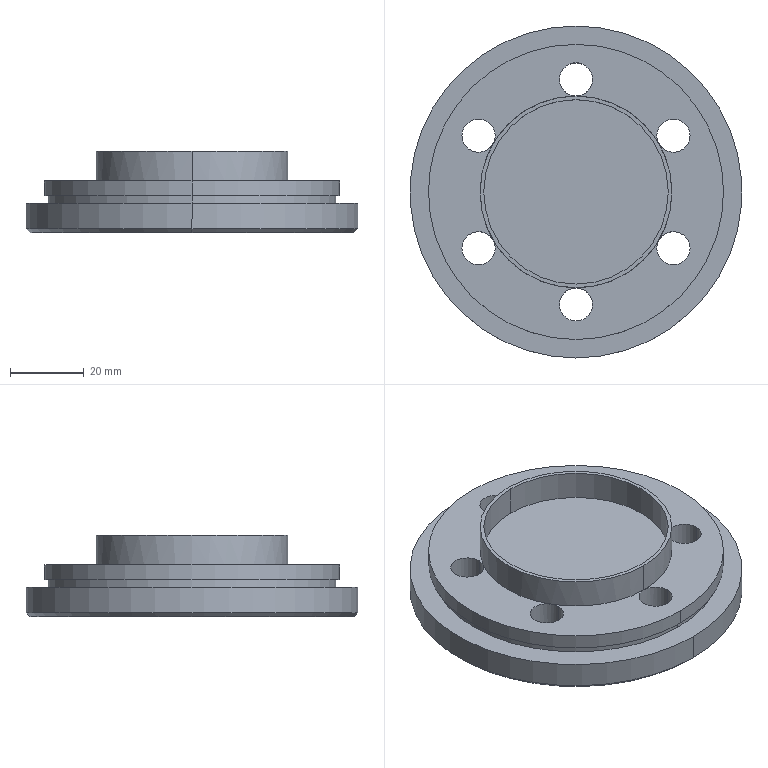Component | SolidWorks | SecondaryEndCover-2 | 1 solid | 33 faces | box 90 x 90 x 22 mm | volume 75360 mm3 | cylinder 22 | plane 7 | cone 2 | torus 2 | commonest cylinder face diameters 9 x12 50 x2 52 x2 78 x2 90 x2 80 x2
build123d program:
from build123d import *

# Parameters (mm, degrees)
SKETCH2_R                  = 26
BOSS_EXTRUDE1_DEPTH        = 8
F_8_5_8_5_DIAMETER_HOLE1_D = 9
CIRPATTERN2_COUNT          = 6
CHAMFER1_SIZE              = 1
SKETCH8_R                  = 25
CUT_EXTRUDE1_DEPTH         = 8


with BuildPart() as part:
    # Sketch1 → Revolve1 (revolve)
    with BuildSketch(Plane(origin=(0, 0, 0), x_dir=(-1, 0, 0), z_dir=(0, 0, -1)), mode=Mode.PRIVATE) as revolve1_sk:
        Polygon((-6, 40), (-6, 0), (8, 0), (8, 45), (0, 45), (0, 39), (-2, 39), (-2, 40), align=None)
    revolve(revolve1_sk.sketch.rotate(Axis((6, 0, 0), (-1, 0, 0)), 180), axis=Axis((6, 0, 0), (-1, 0, 0)))

    # Sketch2 → Boss-Extrude1 (add)
    with BuildSketch(Plane(origin=(6, 0, 0), x_dir=(0, 0, -1), z_dir=(1, 0, 0))):
        with Locations(Location((0, 0, 0), (0, 0, 90))):
            Circle(SKETCH2_R)
    extrude(amount=BOSS_EXTRUDE1_DEPTH)

    # Sketch5 → Cut-Revolve2 (revolve, cut)
    with BuildSketch(Plane(origin=(0, 0, 0), x_dir=(-1, 0, 0), z_dir=(0, 0, -1)), mode=Mode.PRIVATE) as cut_revolve2_sk:
        with BuildLine():
            Line((7, 17), (7, 0))
            Line((7, 0), (8, 0))
            Line((8, 0), (8, 18))
            ThreePointArc((8, 18), (7.293, 17.707), (7, 17))
        make_face()
    revolve(cut_revolve2_sk.sketch.rotate(Axis((-4.998, 0, 0), (-1, 0, 0)), 180), axis=Axis((-4.998, 0, 0), (-1, 0, 0)), mode=Mode.SUBTRACT)

    # 8.5 _8.5_ Diameter Hole1 (through all)
    with Locations(Plane.ZY.offset(8)):
        with Locations((0, 30.5)):
            f_8_5_8_5_diameter_hole1 = Hole(F_8_5_8_5_DIAMETER_HOLE1_D / 2)

    # CirPattern2: 8.5 _8.5_ Diameter Hole1 ×6 about axis
    cirpattern2_axis = Axis((0, 0, 0), (1, 0, 0))
    for i in range(1, CIRPATTERN2_COUNT):
        add(f_8_5_8_5_diameter_hole1.rotate(cirpattern2_axis, i * 360 / CIRPATTERN2_COUNT), mode=Mode.SUBTRACT)

    # Chamfer1
    chamfer1_edges = [part.edges().sort_by_distance(p)[0] for p in [
        (-8, 45, 0),
    ]]
    chamfer(chamfer1_edges, length=CHAMFER1_SIZE)

    # Sketch8 → Cut-Extrude1 (cut)
    with BuildSketch(Plane(origin=(14, 0, 0), x_dir=(0, 0, -1), z_dir=(1, 0, 0))):
        with Locations(Location((0, 0, 0), (0, 0, 90))):
            Circle(SKETCH8_R)
    extrude(amount=-CUT_EXTRUDE1_DEPTH, mode=Mode.SUBTRACT)


solid = part.part

# Placed as in the assembly
solid = solid.moved(Location((-225, 0, -153), (0, -90, 0)))
STEP:
#1=COLOUR_RGB('',0.7922,0.8196,0.9333);
#2=FILL_AREA_STYLE_COLOUR('',#1);
#3=FILL_AREA_STYLE('',(#2));
#4=SURFACE_STYLE_FILL_AREA(#3);
#5=SURFACE_SIDE_STYLE('',(#4));
#6=SURFACE_STYLE_USAGE(.BOTH.,#5);
#7=PRESENTATION_STYLE_ASSIGNMENT((#6));
#8=CARTESIAN_POINT('',(-8.858,-0.9843,-5.787));
#9=VERTEX_POINT('',#8);
#10=CARTESIAN_POINT('',(-8.858,0.9843,-5.787));
#11=VERTEX_POINT('',#10);
#12=CARTESIAN_POINT('',(-8.858,-0.,-5.787));
#13=DIRECTION('',(0.,-0.,1.));
#14=DIRECTION('',(0.,1.,0.));
#15=AXIS2_PLACEMENT_3D('',#12,#13,#14);
#16=CIRCLE('',#15,0.9843);
#17=EDGE_CURVE('',#9,#11,#16,.T.);
#18=ORIENTED_EDGE('',*,*,#17,.F.);
#19=CARTESIAN_POINT('',(-8.858,-0.9843,-5.472));
#20=VERTEX_POINT('',#19);
#21=CARTESIAN_POINT('',(-8.858,-0.9843,-5.787));
#22=DIRECTION('',(0.,-0.,1.));
#23=VECTOR('',#22,39.37);
#24=LINE('',#21,#23);
#25=EDGE_CURVE('',#9,#20,#24,.T.);
#26=ORIENTED_EDGE('',*,*,#25,.T.);
#27=CARTESIAN_POINT('',(-8.858,0.9843,-5.472));
#28=VERTEX_POINT('',#27);
#29=CARTESIAN_POINT('',(-8.858,-0.,-5.472));
#30=DIRECTION('',(0.,-0.,1.));
#31=DIRECTION('',(0.,1.,0.));
#32=AXIS2_PLACEMENT_3D('',#29,#30,#31);
#33=CIRCLE('',#32,0.9843);
#34=EDGE_CURVE('',#20,#28,#33,.T.);
#35=ORIENTED_EDGE('',*,*,#34,.T.);
#36=CARTESIAN_POINT('',(-8.858,0.9843,-5.787));
#37=DIRECTION('',(0.,-0.,1.));
#38=VECTOR('',#37,39.37);
#39=LINE('',#36,#38);
#40=EDGE_CURVE('',#11,#28,#39,.T.);
#41=ORIENTED_EDGE('',*,*,#40,.F.);
#42=EDGE_LOOP('',(#18,#26,#35,#41));
#43=FACE_OUTER_BOUND('',#42,.T.);
#44=CARTESIAN_POINT('',(-8.858,-0.,-5.787));
#45=DIRECTION('',(0.,-0.,1.));
#46=DIRECTION('',(0.,1.,0.));
#47=AXIS2_PLACEMENT_3D('',#44,#45,#46);
#48=CYLINDRICAL_SURFACE('',#47,0.9843);
#49=ADVANCED_FACE('',(#43),#48,.F.);
#50=CARTESIAN_POINT('',(-8.858,-1.732,-6.339));
#51=VERTEX_POINT('',#50);
#52=CARTESIAN_POINT('',(-8.858,1.732,-6.339));
#53=VERTEX_POINT('',#52);
#54=CARTESIAN_POINT('',(-8.858,-0.,-6.339));
#55=DIRECTION('',(-0.,0.,-1.));
#56=DIRECTION('',(0.,-1.,0.));
#57=AXIS2_PLACEMENT_3D('',#54,#55,#56);
#58=CIRCLE('',#57,1.732);
#59=EDGE_CURVE('',#51,#53,#58,.T.);
#60=ORIENTED_EDGE('',*,*,#59,.F.);
#61=CARTESIAN_POINT('',(-8.858,-1.772,-6.299));
#62=VERTEX_POINT('',#61);
#63=CARTESIAN_POINT('',(-8.858,-1.732,-6.339));
#64=DIRECTION('',(0.,-0.7071,0.7071));
#65=VECTOR('',#64,39.37);
#66=LINE('',#63,#65);
#67=EDGE_CURVE('',#51,#62,#66,.T.);
#68=ORIENTED_EDGE('',*,*,#67,.T.);
#69=CARTESIAN_POINT('',(-8.858,1.772,-6.299));
#70=VERTEX_POINT('',#69);
#71=CARTESIAN_POINT('',(-8.858,-0.,-6.299));
#72=DIRECTION('',(0.,-0.,1.));
#73=DIRECTION('',(0.,-1.,0.));
#74=AXIS2_PLACEMENT_3D('',#71,#72,#73);
#75=CIRCLE('',#74,1.772);
#76=EDGE_CURVE('',#70,#62,#75,.T.);
#77=ORIENTED_EDGE('',*,*,#76,.F.);
#78=CARTESIAN_POINT('',(-8.858,1.732,-6.339));
#79=DIRECTION('',(0.,0.7071,0.7071));
#80=VECTOR('',#79,39.37);
#81=LINE('',#78,#80);
#82=EDGE_CURVE('',#53,#70,#81,.T.);
#83=ORIENTED_EDGE('',*,*,#82,.F.);
#84=EDGE_LOOP('',(#60,#68,#77,#83));
#85=FACE_OUTER_BOUND('',#84,.T.);
#86=CARTESIAN_POINT('',(-8.858,-0.,-6.339));
#87=DIRECTION('',(0.,-0.,1.));
#88=DIRECTION('',(0.,1.,0.));
#89=AXIS2_PLACEMENT_3D('',#86,#87,#88);
#90=CONICAL_SURFACE('',#89,1.732,0.7854);
#91=ADVANCED_FACE('',(#85),#90,.T.);
#92=CARTESIAN_POINT('',(-9.745,0.5118,-5.787));
#93=VERTEX_POINT('',#92);
#94=CARTESIAN_POINT('',(-9.721,0.6004,-5.787));
#95=VERTEX_POINT('',#94);
#96=CARTESIAN_POINT('',(-9.898,0.6004,-5.787));
#97=DIRECTION('',(0.,-0.,1.));
#98=DIRECTION('',(0.,1.,0.));
#99=AXIS2_PLACEMENT_3D('',#96,#97,#98);
#100=CIRCLE('',#99,0.1772);
#101=EDGE_CURVE('',#93,#95,#100,.T.);
#102=ORIENTED_EDGE('',*,*,#101,.T.);
#103=CARTESIAN_POINT('',(-9.721,0.6004,-6.339));
#104=VERTEX_POINT('',#103);
#105=CARTESIAN_POINT('',(-9.721,0.6004,-6.339));
#106=DIRECTION('',(-0.,0.,-1.));
#107=VECTOR('',#106,39.37);
#108=LINE('',#105,#107);
#109=EDGE_CURVE('',#95,#104,#108,.T.);
#110=ORIENTED_EDGE('',*,*,#109,.T.);
#111=CARTESIAN_POINT('',(-10.075,0.6004,-6.339));
#112=VERTEX_POINT('',#111);
#113=CARTESIAN_POINT('',(-9.898,0.6004,-6.339));
#114=DIRECTION('',(-0.,0.,-1.));
#115=DIRECTION('',(-1.,0.,0.));
#116=AXIS2_PLACEMENT_3D('',#113,#114,#115);
#117=CIRCLE('',#116,0.1772);
#118=EDGE_CURVE('',#104,#112,#117,.T.);
#119=ORIENTED_EDGE('',*,*,#118,.T.);
#120=CARTESIAN_POINT('',(-10.075,0.6004,-5.787));
#121=VERTEX_POINT('',#120);
#122=CARTESIAN_POINT('',(-10.075,0.6004,-6.339));
#123=DIRECTION('',(-0.,0.,-1.));
#124=VECTOR('',#123,39.37);
#125=LINE('',#122,#124);
#126=EDGE_CURVE('',#121,#112,#125,.T.);
#127=ORIENTED_EDGE('',*,*,#126,.F.);
#128=CARTESIAN_POINT('',(-9.898,0.6004,-5.787));
#129=DIRECTION('',(0.,-0.,1.));
#130=DIRECTION('',(0.,1.,0.));
#131=AXIS2_PLACEMENT_3D('',#128,#129,#130);
#132=CIRCLE('',#131,0.1772);
#133=EDGE_CURVE('',#121,#93,#132,.T.);
#134=ORIENTED_EDGE('',*,*,#133,.T.);
#135=EDGE_LOOP('',(#102,#110,#119,#127,#134));
#136=FACE_OUTER_BOUND('',#135,.T.);
#137=CARTESIAN_POINT('',(-9.898,0.6004,-6.339));
#138=DIRECTION('',(-0.,0.,-1.));
#139=DIRECTION('',(-1.,0.,0.));
#140=AXIS2_PLACEMENT_3D('',#137,#138,#139);
#141=CYLINDRICAL_SURFACE('',#140,0.1772);
#142=ADVANCED_FACE('',(#136),#141,.F.);
#143=CARTESIAN_POINT('',(-10.075,-0.6004,-5.787));
#144=VERTEX_POINT('',#143);
#145=CARTESIAN_POINT('',(-9.721,-0.6004,-5.787));
#146=VERTEX_POINT('',#145);
#147=CARTESIAN_POINT('',(-9.898,-0.6004,-5.787));
#148=DIRECTION('',(0.,-0.,1.));
#149=DIRECTION('',(0.,1.,0.));
#150=AXIS2_PLACEMENT_3D('',#147,#148,#149);
#151=CIRCLE('',#150,0.1772);
#152=EDGE_CURVE('',#144,#146,#151,.T.);
#153=ORIENTED_EDGE('',*,*,#152,.T.);
#154=CARTESIAN_POINT('',(-9.721,-0.6004,-6.339));
#155=VERTEX_POINT('',#154);
#156=CARTESIAN_POINT('',(-9.721,-0.6004,-6.339));
#157=DIRECTION('',(-0.,0.,-1.));
#158=VECTOR('',#157,39.37);
#159=LINE('',#156,#158);
#160=EDGE_CURVE('',#146,#155,#159,.T.);
#161=ORIENTED_EDGE('',*,*,#160,.T.);
#162=CARTESIAN_POINT('',(-10.075,-0.6004,-6.339));
#163=VERTEX_POINT('',#162);
#164=CARTESIAN_POINT('',(-9.898,-0.6004,-6.339));
#165=DIRECTION('',(-0.,0.,-1.));
#166=DIRECTION('',(-1.,0.,0.));
#167=AXIS2_PLACEMENT_3D('',#164,#165,#166);
#168=CIRCLE('',#167,0.1772);
#169=EDGE_CURVE('',#155,#163,#168,.T.);
#170=ORIENTED_EDGE('',*,*,#169,.T.);
#171=CARTESIAN_POINT('',(-10.075,-0.6004,-6.339));
#172=DIRECTION('',(-0.,0.,-1.));
#173=VECTOR('',#172,39.37);
#174=LINE('',#171,#173);
#175=EDGE_CURVE('',#144,#163,#174,.T.);
#176=ORIENTED_EDGE('',*,*,#175,.F.);
#177=EDGE_LOOP('',(#153,#161,#170,#176));
#178=FACE_OUTER_BOUND('',#177,.T.);
#179=CARTESIAN_POINT('',(-9.898,-0.6004,-6.339));
#180=DIRECTION('',(-0.,0.,-1.));
#181=DIRECTION('',(-1.,0.,0.));
#182=AXIS2_PLACEMENT_3D('',#179,#180,#181);
#183=CYLINDRICAL_SURFACE('',#182,0.1772);
#184=ADVANCED_FACE('',(#178),#183,.F.);
#185=CARTESIAN_POINT('',(-9.035,-1.201,-5.787));
#186=VERTEX_POINT('',#185);
#187=CARTESIAN_POINT('',(-8.681,-1.201,-5.787));
#188=VERTEX_POINT('',#187);
#189=CARTESIAN_POINT('',(-8.858,-1.201,-5.787));
#190=DIRECTION('',(0.,-0.,1.));
#191=DIRECTION('',(0.,1.,0.));
#192=AXIS2_PLACEMENT_3D('',#189,#190,#191);
#193=CIRCLE('',#192,0.1772);
#194=EDGE_CURVE('',#186,#188,#193,.T.);
#195=ORIENTED_EDGE('',*,*,#194,.T.);
#196=CARTESIAN_POINT('',(-8.681,-1.201,-6.339));
#197=VERTEX_POINT('',#196);
#198=CARTESIAN_POINT('',(-8.681,-1.201,-6.339));
#199=DIRECTION('',(-0.,0.,-1.));
#200=VECTOR('',#199,39.37);
#201=LINE('',#198,#200);
#202=EDGE_CURVE('',#188,#197,#201,.T.);
#203=ORIENTED_EDGE('',*,*,#202,.T.);
#204=CARTESIAN_POINT('',(-9.035,-1.201,-6.339));
#205=VERTEX_POINT('',#204);
#206=CARTESIAN_POINT('',(-8.858,-1.201,-6.339));
#207=DIRECTION('',(-0.,0.,-1.));
#208=DIRECTION('',(-1.,0.,0.));
#209=AXIS2_PLACEMENT_3D('',#206,#207,#208);
#210=CIRCLE('',#209,0.1772);
#211=EDGE_CURVE('',#197,#205,#210,.T.);
#212=ORIENTED_EDGE('',*,*,#211,.T.);
#213=CARTESIAN_POINT('',(-9.035,-1.201,-6.339));
#214=DIRECTION('',(-0.,0.,-1.));
#215=VECTOR('',#214,39.37);
#216=LINE('',#213,#215);
#217=EDGE_CURVE('',#186,#205,#216,.T.);
#218=ORIENTED_EDGE('',*,*,#217,.F.);
#219=EDGE_LOOP('',(#195,#203,#212,#218));
#220=FACE_OUTER_BOUND('',#219,.T.);
#221=CARTESIAN_POINT('',(-8.858,-1.201,-6.339));
#222=DIRECTION('',(-0.,0.,-1.));
#223=DIRECTION('',(-1.,0.,0.));
#224=AXIS2_PLACEMENT_3D('',#221,#222,#223);
#225=CYLINDRICAL_SURFACE('',#224,0.1772);
#226=ADVANCED_FACE('',(#220),#225,.F.);
#227=CARTESIAN_POINT('',(-7.996,-0.6004,-5.787));
#228=VERTEX_POINT('',#227);
#229=CARTESIAN_POINT('',(-7.641,-0.6004,-5.787));
#230=VERTEX_POINT('',#229);
#231=CARTESIAN_POINT('',(-7.818,-0.6004,-5.787));
#232=DIRECTION('',(0.,-0.,1.));
#233=DIRECTION('',(0.,1.,0.));
#234=AXIS2_PLACEMENT_3D('',#231,#232,#233);
#235=CIRCLE('',#234,0.1772);
#236=EDGE_CURVE('',#228,#230,#235,.T.);
#237=ORIENTED_EDGE('',*,*,#236,.T.);
#238=CARTESIAN_POINT('',(-7.641,-0.6004,-6.339));
#239=VERTEX_POINT('',#238);
#240=CARTESIAN_POINT('',(-7.641,-0.6004,-6.339));
#241=DIRECTION('',(-0.,0.,-1.));
#242=VECTOR('',#241,39.37);
#243=LINE('',#240,#242);
#244=EDGE_CURVE('',#230,#239,#243,.T.);
#245=ORIENTED_EDGE('',*,*,#244,.T.);
#246=CARTESIAN_POINT('',(-7.996,-0.6004,-6.339));
#247=VERTEX_POINT('',#246);
#248=CARTESIAN_POINT('',(-7.818,-0.6004,-6.339));
#249=DIRECTION('',(-0.,0.,-1.));
#250=DIRECTION('',(-1.,0.,0.));
#251=AXIS2_PLACEMENT_3D('',#248,#249,#250);
#252=CIRCLE('',#251,0.1772);
#253=EDGE_CURVE('',#239,#247,#252,.T.);
#254=ORIENTED_EDGE('',*,*,#253,.T.);
#255=CARTESIAN_POINT('',(-7.996,-0.6004,-6.339));
#256=DIRECTION('',(-0.,0.,-1.));
#257=VECTOR('',#256,39.37);
#258=LINE('',#255,#257);
#259=EDGE_CURVE('',#228,#247,#258,.T.);
#260=ORIENTED_EDGE('',*,*,#259,.F.);
#261=EDGE_LOOP('',(#237,#245,#254,#260));
#262=FACE_OUTER_BOUND('',#261,.T.);
#263=CARTESIAN_POINT('',(-7.818,-0.6004,-6.339));
#264=DIRECTION('',(-0.,0.,-1.));
#265=DIRECTION('',(-1.,0.,0.));
#266=AXIS2_PLACEMENT_3D('',#263,#264,#265);
#267=CYLINDRICAL_SURFACE('',#266,0.1772);
#268=ADVANCED_FACE('',(#262),#267,.F.);
#269=CARTESIAN_POINT('',(-7.972,0.5118,-5.787));
#270=VERTEX_POINT('',#269);
#271=CARTESIAN_POINT('',(-7.641,0.6004,-5.787));
#272=VERTEX_POINT('',#271);
#273=CARTESIAN_POINT('',(-7.818,0.6004,-5.787));
#274=DIRECTION('',(0.,-0.,1.));
#275=DIRECTION('',(0.,1.,0.));
#276=AXIS2_PLACEMENT_3D('',#273,#274,#275);
#277=CIRCLE('',#276,0.1772);
#278=EDGE_CURVE('',#270,#272,#277,.T.);
#279=ORIENTED_EDGE('',*,*,#278,.T.);
#280=CARTESIAN_POINT('',(-7.641,0.6004,-6.339));
#281=VERTEX_POINT('',#280);
#282=CARTESIAN_POINT('',(-7.641,0.6004,-6.339));
#283=DIRECTION('',(-0.,0.,-1.));
#284=VECTOR('',#283,39.37);
#285=LINE('',#282,#284);
#286=EDGE_CURVE('',#272,#281,#285,.T.);
#287=ORIENTED_EDGE('',*,*,#286,.T.);
#288=CARTESIAN_POINT('',(-7.996,0.6004,-6.339));
#289=VERTEX_POINT('',#288);
#290=CARTESIAN_POINT('',(-7.818,0.6004,-6.339));
#291=DIRECTION('',(-0.,0.,-1.));
#292=DIRECTION('',(-1.,0.,0.));
#293=AXIS2_PLACEMENT_3D('',#290,#291,#292);
#294=CIRCLE('',#293,0.1772);
#295=EDGE_CURVE('',#281,#289,#294,.T.);
#296=ORIENTED_EDGE('',*,*,#295,.T.);
#297=CARTESIAN_POINT('',(-7.996,0.6004,-5.787));
#298=VERTEX_POINT('',#297);
#299=CARTESIAN_POINT('',(-7.996,0.6004,-6.339));
#300=DIRECTION('',(-0.,0.,-1.));
#301=VECTOR('',#300,39.37);
#302=LINE('',#299,#301);
#303=EDGE_CURVE('',#298,#289,#302,.T.);
#304=ORIENTED_EDGE('',*,*,#303,.F.);
#305=CARTESIAN_POINT('',(-7.818,0.6004,-5.787));
#306=DIRECTION('',(0.,-0.,1.));
#307=DIRECTION('',(0.,1.,0.));
#308=AXIS2_PLACEMENT_3D('',#305,#306,#307);
#309=CIRCLE('',#308,0.1772);
#310=EDGE_CURVE('',#298,#270,#309,.T.);
#311=ORIENTED_EDGE('',*,*,#310,.T.);
#312=EDGE_LOOP('',(#279,#287,#296,#304,#311));
#313=FACE_OUTER_BOUND('',#312,.T.);
#314=CARTESIAN_POINT('',(-7.818,0.6004,-6.339));
#315=DIRECTION('',(-0.,0.,-1.));
#316=DIRECTION('',(-1.,0.,0.));
#317=AXIS2_PLACEMENT_3D('',#314,#315,#316);
#318=CYLINDRICAL_SURFACE('',#317,0.1772);
#319=ADVANCED_FACE('',(#313),#318,.F.);
#320=CARTESIAN_POINT('',(-8.858,1.024,-5.787));
#321=VERTEX_POINT('',#320);
#322=CARTESIAN_POINT('',(-8.681,1.201,-5.787));
#323=VERTEX_POINT('',#322);
#324=CARTESIAN_POINT('',(-8.858,1.201,-5.787));
#325=DIRECTION('',(0.,-0.,1.));
#326=DIRECTION('',(0.,1.,0.));
#327=AXIS2_PLACEMENT_3D('',#324,#325,#326);
#328=CIRCLE('',#327,0.1772);
#329=EDGE_CURVE('',#321,#323,#328,.T.);
#330=ORIENTED_EDGE('',*,*,#329,.T.);
#331=CARTESIAN_POINT('',(-8.681,1.201,-6.339));
#332=VERTEX_POINT('',#331);
#333=CARTESIAN_POINT('',(-8.681,1.201,-6.339));
#334=DIRECTION('',(-0.,0.,-1.));
#335=VECTOR('',#334,39.37);
#336=LINE('',#333,#335);
#337=EDGE_CURVE('',#323,#332,#336,.T.);
#338=ORIENTED_EDGE('',*,*,#337,.T.);
#339=CARTESIAN_POINT('',(-9.035,1.201,-6.339));
#340=VERTEX_POINT('',#339);
#341=CARTESIAN_POINT('',(-8.858,1.201,-6.339));
#342=DIRECTION('',(-0.,0.,-1.));
#343=DIRECTION('',(-1.,0.,0.));
#344=AXIS2_PLACEMENT_3D('',#341,#342,#343);
#345=CIRCLE('',#344,0.1772);
#346=EDGE_CURVE('',#332,#340,#345,.T.);
#347=ORIENTED_EDGE('',*,*,#346,.T.);
#348=CARTESIAN_POINT('',(-9.035,1.201,-5.787));
#349=VERTEX_POINT('',#348);
#350=CARTESIAN_POINT('',(-9.035,1.201,-6.339));
#351=DIRECTION('',(-0.,0.,-1.));
#352=VECTOR('',#351,39.37);
#353=LINE('',#350,#352);
#354=EDGE_CURVE('',#349,#340,#353,.T.);
#355=ORIENTED_EDGE('',*,*,#354,.F.);
#356=CARTESIAN_POINT('',(-8.858,1.201,-5.787));
#357=DIRECTION('',(0.,-0.,1.));
#358=DIRECTION('',(0.,1.,0.));
#359=AXIS2_PLACEMENT_3D('',#356,#357,#358);
#360=CIRCLE('',#359,0.1772);
#361=EDGE_CURVE('',#349,#321,#360,.T.);
#362=ORIENTED_EDGE('',*,*,#361,.T.);
#363=EDGE_LOOP('',(#330,#338,#347,#355,#362));
#364=FACE_OUTER_BOUND('',#363,.T.);
#365=CARTESIAN_POINT('',(-8.858,1.201,-6.339));
#366=DIRECTION('',(-0.,0.,-1.));
#367=DIRECTION('',(-1.,0.,0.));
#368=AXIS2_PLACEMENT_3D('',#365,#366,#367);
#369=CYLINDRICAL_SURFACE('',#368,0.1772);
#370=ADVANCED_FACE('',(#364),#369,.F.);
#371=CARTESIAN_POINT('',(-8.858,0.6693,-6.299));
#372=VERTEX_POINT('',#371);
#373=CARTESIAN_POINT('',(-8.858,-0.6693,-6.299));
#374=VERTEX_POINT('',#373);
#375=CARTESIAN_POINT('',(-8.858,-0.,-6.299));
#376=DIRECTION('',(-0.,0.,-1.));
#377=DIRECTION('',(0.,-1.,0.));
#378=AXIS2_PLACEMENT_3D('',#375,#376,#377);
#379=CIRCLE('',#378,0.6693);
#380=EDGE_CURVE('',#372,#374,#379,.T.);
#381=ORIENTED_EDGE('',*,*,#380,.F.);
#382=CARTESIAN_POINT('',(-8.858,0.7087,-6.339));
#383=VERTEX_POINT('',#382);
#384=CARTESIAN_POINT('',(-8.858,0.6693,-6.339));
#385=DIRECTION('',(-1.,-0.,0.));
#386=DIRECTION('',(0.,0.,1.));
#387=AXIS2_PLACEMENT_3D('',#384,#385,#386);
#388=CIRCLE('',#387,0.03937);
#389=EDGE_CURVE('',#372,#383,#388,.T.);
#390=ORIENTED_EDGE('',*,*,#389,.T.);
#391=CARTESIAN_POINT('',(-8.858,-0.7087,-6.339));
#392=VERTEX_POINT('',#391);
#393=CARTESIAN_POINT('',(-8.858,-0.,-6.339));
#394=DIRECTION('',(-0.,0.,-1.));
#395=DIRECTION('',(0.,-1.,0.));
#396=AXIS2_PLACEMENT_3D('',#393,#394,#395);
#397=CIRCLE('',#396,0.7087);
#398=EDGE_CURVE('',#383,#392,#397,.T.);
#399=ORIENTED_EDGE('',*,*,#398,.T.);
#400=CARTESIAN_POINT('',(-8.858,-0.6693,-6.339));
#401=DIRECTION('',(1.,0.,-0.));
#402=DIRECTION('',(0.,0.,-1.));
#403=AXIS2_PLACEMENT_3D('',#400,#401,#402);
#404=CIRCLE('',#403,0.03937);
#405=EDGE_CURVE('',#374,#392,#404,.T.);
#406=ORIENTED_EDGE('',*,*,#405,.F.);
#407=EDGE_LOOP('',(#381,#390,#399,#406));
#408=FACE_OUTER_BOUND('',#407,.T.);
#409=CARTESIAN_POINT('',(-8.858,-0.,-6.339));
#410=DIRECTION('',(-0.,0.,-1.));
#411=DIRECTION('',(-0.,-1.,-0.));
#412=AXIS2_PLACEMENT_3D('',#409,#410,#411);
#413=TOROIDAL_SURFACE('',#412,0.6693,0.03937);
#414=ADVANCED_FACE('',(#408),#413,.F.);
#415=CARTESIAN_POINT('',(-8.858,1.024,-5.472));
#416=VERTEX_POINT('',#415);
#417=CARTESIAN_POINT('',(-8.858,-1.024,-5.472));
#418=VERTEX_POINT('',#417);
#419=CARTESIAN_POINT('',(-8.858,-0.,-5.472));
#420=DIRECTION('',(0.,-0.,1.));
#421=DIRECTION('',(0.,1.,0.));
#422=AXIS2_PLACEMENT_3D('',#419,#420,#421);
#423=CIRCLE('',#422,1.024);
#424=EDGE_CURVE('',#416,#418,#423,.T.);
#425=ORIENTED_EDGE('',*,*,#424,.F.);
#426=CARTESIAN_POINT('',(-8.858,1.024,-5.472));
#427=DIRECTION('',(-0.,0.,-1.));
#428=VECTOR('',#427,39.37);
#429=LINE('',#426,#428);
#430=EDGE_CURVE('',#416,#321,#429,.T.);
#431=ORIENTED_EDGE('',*,*,#430,.T.);
#432=CARTESIAN_POINT('',(-8.858,-0.,-5.787));
#433=DIRECTION('',(0.,-0.,1.));
#434=DIRECTION('',(0.,1.,0.));
#435=AXIS2_PLACEMENT_3D('',#432,#433,#434);
#436=CIRCLE('',#435,1.024);
#437=EDGE_CURVE('',#321,#93,#436,.T.);
#438=ORIENTED_EDGE('',*,*,#437,.T.);
#439=CARTESIAN_POINT('',(-9.745,-0.5118,-5.787));
#440=VERTEX_POINT('',#439);
#441=CARTESIAN_POINT('',(-8.858,-0.,-5.787));
#442=DIRECTION('',(0.,-0.,1.));
#443=DIRECTION('',(0.,1.,0.));
#444=AXIS2_PLACEMENT_3D('',#441,#442,#443);
#445=CIRCLE('',#444,1.024);
#446=EDGE_CURVE('',#93,#440,#445,.T.);
#447=ORIENTED_EDGE('',*,*,#446,.T.);
#448=CARTESIAN_POINT('',(-8.858,-1.024,-5.787));
#449=VERTEX_POINT('',#448);
#450=CARTESIAN_POINT('',(-8.858,-0.,-5.787));
#451=DIRECTION('',(0.,-0.,1.));
#452=DIRECTION('',(0.,1.,0.));
#453=AXIS2_PLACEMENT_3D('',#450,#451,#452);
#454=CIRCLE('',#453,1.024);
#455=EDGE_CURVE('',#440,#449,#454,.T.);
#456=ORIENTED_EDGE('',*,*,#455,.T.);
#457=CARTESIAN_POINT('',(-8.858,-1.024,-5.472));
#458=DIRECTION('',(-0.,0.,-1.));
#459=VECTOR('',#458,39.37);
#460=LINE('',#457,#459);
#461=EDGE_CURVE('',#418,#449,#460,.T.);
#462=ORIENTED_EDGE('',*,*,#461,.F.);
#463=EDGE_LOOP('',(#425,#431,#438,#447,#456,#462));
#464=FACE_OUTER_BOUND('',#463,.T.);
#465=CARTESIAN_POINT('',(-8.858,-0.,-5.472));
#466=DIRECTION('',(-0.,0.,-1.));
#467=DIRECTION('',(0.,-1.,0.));
#468=AXIS2_PLACEMENT_3D('',#465,#466,#467);
#469=CYLINDRICAL_SURFACE('',#468,1.024);
#470=ADVANCED_FACE('',(#464),#469,.T.);
#471=CARTESIAN_POINT('',(-8.858,-1.535,-5.945));
#472=VERTEX_POINT('',#471);
#473=CARTESIAN_POINT('',(-8.858,1.535,-5.945));
#474=VERTEX_POINT('',#473);
#475=CARTESIAN_POINT('',(-8.858,-0.,-5.945));
#476=DIRECTION('',(-0.,0.,-1.));
#477=DIRECTION('',(0.,-1.,0.));
#478=AXIS2_PLACEMENT_3D('',#475,#476,#477);
#479=CIRCLE('',#478,1.535);
#480=EDGE_CURVE('',#472,#474,#479,.T.);
#481=ORIENTED_EDGE('',*,*,#480,.T.);
#482=CARTESIAN_POINT('',(-8.858,1.535,-6.024));
#483=VERTEX_POINT('',#482);
#484=CARTESIAN_POINT('',(-8.858,1.535,-5.787));
#485=DIRECTION('',(-0.,0.,-1.));
#486=VECTOR('',#485,39.37);
#487=LINE('',#484,#486);
#488=EDGE_CURVE('',#474,#483,#487,.T.);
#489=ORIENTED_EDGE('',*,*,#488,.T.);
#490=CARTESIAN_POINT('',(-8.858,-1.535,-6.024));
#491=VERTEX_POINT('',#490);
#492=CARTESIAN_POINT('',(-8.858,-0.,-6.024));
#493=DIRECTION('',(-0.,0.,-1.));
#494=DIRECTION('',(0.,-1.,0.));
#495=AXIS2_PLACEMENT_3D('',#492,#493,#494);
#496=CIRCLE('',#495,1.535);
#497=EDGE_CURVE('',#491,#483,#496,.T.);
#498=ORIENTED_EDGE('',*,*,#497,.F.);
#499=CARTESIAN_POINT('',(-8.858,-1.535,-5.787));
#500=DIRECTION('',(-0.,0.,-1.));
#501=VECTOR('',#500,39.37);
#502=LINE('',#499,#501);
#503=EDGE_CURVE('',#472,#491,#502,.T.);
#504=ORIENTED_EDGE('',*,*,#503,.F.);
#505=EDGE_LOOP('',(#481,#489,#498,#504));
#506=FACE_OUTER_BOUND('',#505,.T.);
#507=CARTESIAN_POINT('',(-8.858,-0.,-5.787));
#508=DIRECTION('',(-0.,0.,-1.));
#509=DIRECTION('',(0.,-1.,0.));
#510=AXIS2_PLACEMENT_3D('',#507,#508,#509);
#511=CYLINDRICAL_SURFACE('',#510,1.535);
#512=ADVANCED_FACE('',(#506),#511,.T.);
#513=CARTESIAN_POINT('',(-8.858,-1.772,-6.024));
#514=VERTEX_POINT('',#513);
#515=CARTESIAN_POINT('',(-8.858,1.772,-6.024));
#516=VERTEX_POINT('',#515);
#517=CARTESIAN_POINT('',(-8.858,-0.,-6.024));
#518=DIRECTION('',(-0.,0.,-1.));
#519=DIRECTION('',(0.,-1.,0.));
#520=AXIS2_PLACEMENT_3D('',#517,#518,#519);
#521=CIRCLE('',#520,1.772);
#522=EDGE_CURVE('',#514,#516,#521,.T.);
#523=ORIENTED_EDGE('',*,*,#522,.T.);
#524=CARTESIAN_POINT('',(-8.858,1.772,-5.787));
#525=DIRECTION('',(-0.,0.,-1.));
#526=VECTOR('',#525,39.37);
#527=LINE('',#524,#526);
#528=EDGE_CURVE('',#516,#70,#527,.T.);
#529=ORIENTED_EDGE('',*,*,#528,.T.);
#530=ORIENTED_EDGE('',*,*,#76,.T.);
#531=CARTESIAN_POINT('',(-8.858,-1.772,-5.787));
#532=DIRECTION('',(-0.,0.,-1.));
#533=VECTOR('',#532,39.37);
#534=LINE('',#531,#533);
#535=EDGE_CURVE('',#514,#62,#534,.T.);
#536=ORIENTED_EDGE('',*,*,#535,.F.);
#537=EDGE_LOOP('',(#523,#529,#530,#536));
#538=FACE_OUTER_BOUND('',#537,.T.);
#539=CARTESIAN_POINT('',(-8.858,-0.,-5.787));
#540=DIRECTION('',(-0.,0.,-1.));
#541=DIRECTION('',(0.,-1.,0.));
#542=AXIS2_PLACEMENT_3D('',#539,#540,#541);
#543=CYLINDRICAL_SURFACE('',#542,1.772);
#544=ADVANCED_FACE('',(#538),#543,.T.);
#545=CARTESIAN_POINT('',(-8.858,-1.575,-5.787));
#546=VERTEX_POINT('',#545);
#547=CARTESIAN_POINT('',(-8.858,1.575,-5.787));
#548=VERTEX_POINT('',#547);
#549=CARTESIAN_POINT('',(-8.858,-0.,-5.787));
#550=DIRECTION('',(-0.,0.,-1.));
#551=DIRECTION('',(0.,-1.,0.));
#552=AXIS2_PLACEMENT_3D('',#549,#550,#551);
#553=CIRCLE('',#552,1.575);
#554=EDGE_CURVE('',#546,#548,#553,.T.);
#555=ORIENTED_EDGE('',*,*,#554,.T.);
#556=CARTESIAN_POINT('',(-8.858,1.575,-5.945));
#557=VERTEX_POINT('',#556);
#558=CARTESIAN_POINT('',(-8.858,1.575,-5.787));
#559=DIRECTION('',(-0.,0.,-1.));
#560=VECTOR('',#559,39.37);
#561=LINE('',#558,#560);
#562=EDGE_CURVE('',#548,#557,#561,.T.);
#563=ORIENTED_EDGE('',*,*,#562,.T.);
#564=CARTESIAN_POINT('',(-8.858,-1.575,-5.945));
#565=VERTEX_POINT('',#564);
#566=CARTESIAN_POINT('',(-8.858,-0.,-5.945));
#567=DIRECTION('',(-0.,0.,-1.));
#568=DIRECTION('',(0.,-1.,0.));
#569=AXIS2_PLACEMENT_3D('',#566,#567,#568);
#570=CIRCLE('',#569,1.575);
#571=EDGE_CURVE('',#565,#557,#570,.T.);
#572=ORIENTED_EDGE('',*,*,#571,.F.);
#573=CARTESIAN_POINT('',(-8.858,-1.575,-5.787));
#574=DIRECTION('',(-0.,0.,-1.));
#575=VECTOR('',#574,39.37);
#576=LINE('',#573,#575);
#577=EDGE_CURVE('',#546,#565,#576,.T.);
#578=ORIENTED_EDGE('',*,*,#577,.F.);
#579=EDGE_LOOP('',(#555,#563,#572,#578));
#580=FACE_OUTER_BOUND('',#579,.T.);
#581=CARTESIAN_POINT('',(-8.858,-0.,-5.787));
#582=DIRECTION('',(-0.,0.,-1.));
#583=DIRECTION('',(0.,-1.,0.));
#584=AXIS2_PLACEMENT_3D('',#581,#582,#583);
#585=CYLINDRICAL_SURFACE('',#584,1.575);
#586=ADVANCED_FACE('',(#580),#585,.T.);
#587=ORIENTED_EDGE('',*,*,#562,.F.);
#588=CARTESIAN_POINT('',(-8.858,-0.,-5.787));
#589=DIRECTION('',(-0.,0.,-1.));
#590=DIRECTION('',(0.,-1.,0.));
#591=AXIS2_PLACEMENT_3D('',#588,#589,#590);
#592=CIRCLE('',#591,1.575);
#593=EDGE_CURVE('',#548,#546,#592,.T.);
#594=ORIENTED_EDGE('',*,*,#593,.T.);
#595=ORIENTED_EDGE('',*,*,#577,.T.);
#596=CARTESIAN_POINT('',(-8.858,-0.,-5.945));
#597=DIRECTION('',(-0.,0.,-1.));
#598=DIRECTION('',(0.,-1.,0.));
#599=AXIS2_PLACEMENT_3D('',#596,#597,#598);
#600=CIRCLE('',#599,1.575);
#601=EDGE_CURVE('',#557,#565,#600,.T.);
#602=ORIENTED_EDGE('',*,*,#601,.F.);
#603=EDGE_LOOP('',(#587,#594,#595,#602));
#604=FACE_OUTER_BOUND('',#603,.T.);
#605=CARTESIAN_POINT('',(-8.858,-0.,-5.787));
#606=DIRECTION('',(-0.,0.,-1.));
#607=DIRECTION('',(0.,-1.,0.));
#608=AXIS2_PLACEMENT_3D('',#605,#606,#607);
#609=CYLINDRICAL_SURFACE('',#608,1.575);
#610=ADVANCED_FACE('',(#604),#609,.T.);
#611=ORIENTED_EDGE('',*,*,#446,.F.);
#612=ORIENTED_EDGE('',*,*,#133,.F.);
#613=CARTESIAN_POINT('',(-9.898,0.6004,-5.787));
#614=DIRECTION('',(0.,-0.,1.));
#615=DIRECTION('',(0.,1.,0.));
#616=AXIS2_PLACEMENT_3D('',#613,#614,#615);
#617=CIRCLE('',#616,0.1772);
#618=EDGE_CURVE('',#95,#121,#617,.T.);
#619=ORIENTED_EDGE('',*,*,#618,.F.);
#620=ORIENTED_EDGE('',*,*,#101,.F.);
#621=ORIENTED_EDGE('',*,*,#437,.F.);
#622=ORIENTED_EDGE('',*,*,#361,.F.);
#623=CARTESIAN_POINT('',(-8.858,1.201,-5.787));
#624=DIRECTION('',(0.,-0.,1.));
#625=DIRECTION('',(0.,1.,0.));
#626=AXIS2_PLACEMENT_3D('',#623,#624,#625);
#627=CIRCLE('',#626,0.1772);
#628=EDGE_CURVE('',#323,#349,#627,.T.);
#629=ORIENTED_EDGE('',*,*,#628,.F.);
#630=ORIENTED_EDGE('',*,*,#329,.F.);
#631=CARTESIAN_POINT('',(-8.858,-0.,-5.787));
#632=DIRECTION('',(0.,-0.,1.));
#633=DIRECTION('',(0.,1.,0.));
#634=AXIS2_PLACEMENT_3D('',#631,#632,#633);
#635=CIRCLE('',#634,1.024);
#636=EDGE_CURVE('',#270,#321,#635,.T.);
#637=ORIENTED_EDGE('',*,*,#636,.F.);
#638=ORIENTED_EDGE('',*,*,#310,.F.);
#639=CARTESIAN_POINT('',(-7.818,0.6004,-5.787));
#640=DIRECTION('',(0.,-0.,1.));
#641=DIRECTION('',(0.,1.,0.));
#642=AXIS2_PLACEMENT_3D('',#639,#640,#641);
#643=CIRCLE('',#642,0.1772);
#644=EDGE_CURVE('',#272,#298,#643,.T.);
#645=ORIENTED_EDGE('',*,*,#644,.F.);
#646=ORIENTED_EDGE('',*,*,#278,.F.);
#647=CARTESIAN_POINT('',(-7.972,-0.5118,-5.787));
#648=VERTEX_POINT('',#647);
#649=CARTESIAN_POINT('',(-8.858,-0.,-5.787));
#650=DIRECTION('',(0.,-0.,1.));
#651=DIRECTION('',(0.,1.,0.));
#652=AXIS2_PLACEMENT_3D('',#649,#650,#651);
#653=CIRCLE('',#652,1.024);
#654=EDGE_CURVE('',#648,#270,#653,.T.);
#655=ORIENTED_EDGE('',*,*,#654,.F.);
#656=CARTESIAN_POINT('',(-7.818,-0.6004,-5.787));
#657=DIRECTION('',(0.,-0.,1.));
#658=DIRECTION('',(0.,1.,0.));
#659=AXIS2_PLACEMENT_3D('',#656,#657,#658);
#660=CIRCLE('',#659,0.1772);
#661=EDGE_CURVE('',#230,#648,#660,.T.);
#662=ORIENTED_EDGE('',*,*,#661,.F.);
#663=ORIENTED_EDGE('',*,*,#236,.F.);
#664=CARTESIAN_POINT('',(-7.818,-0.6004,-5.787));
#665=DIRECTION('',(0.,-0.,1.));
#666=DIRECTION('',(0.,1.,0.));
#667=AXIS2_PLACEMENT_3D('',#664,#665,#666);
#668=CIRCLE('',#667,0.1772);
#669=EDGE_CURVE('',#648,#228,#668,.T.);
#670=ORIENTED_EDGE('',*,*,#669,.F.);
#671=CARTESIAN_POINT('',(-8.858,-0.,-5.787));
#672=DIRECTION('',(0.,-0.,1.));
#673=DIRECTION('',(0.,1.,0.));
#674=AXIS2_PLACEMENT_3D('',#671,#672,#673);
#675=CIRCLE('',#674,1.024);
#676=EDGE_CURVE('',#449,#648,#675,.T.);
#677=ORIENTED_EDGE('',*,*,#676,.F.);
#678=CARTESIAN_POINT('',(-8.858,-1.201,-5.787));
#679=DIRECTION('',(0.,-0.,1.));
#680=DIRECTION('',(0.,1.,0.));
#681=AXIS2_PLACEMENT_3D('',#678,#679,#680);
#682=CIRCLE('',#681,0.1772);
#683=EDGE_CURVE('',#188,#449,#682,.T.);
#684=ORIENTED_EDGE('',*,*,#683,.F.);
#685=ORIENTED_EDGE('',*,*,#194,.F.);
#686=CARTESIAN_POINT('',(-8.858,-1.201,-5.787));
#687=DIRECTION('',(0.,-0.,1.));
#688=DIRECTION('',(0.,1.,0.));
#689=AXIS2_PLACEMENT_3D('',#686,#687,#688);
#690=CIRCLE('',#689,0.1772);
#691=EDGE_CURVE('',#449,#186,#690,.T.);
#692=ORIENTED_EDGE('',*,*,#691,.F.);
#693=ORIENTED_EDGE('',*,*,#455,.F.);
#694=CARTESIAN_POINT('',(-9.898,-0.6004,-5.787));
#695=DIRECTION('',(0.,-0.,1.));
#696=DIRECTION('',(0.,1.,0.));
#697=AXIS2_PLACEMENT_3D('',#694,#695,#696);
#698=CIRCLE('',#697,0.1772);
#699=EDGE_CURVE('',#146,#440,#698,.T.);
#700=ORIENTED_EDGE('',*,*,#699,.F.);
#701=ORIENTED_EDGE('',*,*,#152,.F.);
#702=CARTESIAN_POINT('',(-9.898,-0.6004,-5.787));
#703=DIRECTION('',(0.,-0.,1.));
#704=DIRECTION('',(0.,1.,0.));
#705=AXIS2_PLACEMENT_3D('',#702,#703,#704);
#706=CIRCLE('',#705,0.1772);
#707=EDGE_CURVE('',#440,#144,#706,.T.);
#708=ORIENTED_EDGE('',*,*,#707,.F.);
#709=EDGE_LOOP('',(#611,#612,#619,#620,#621,#622,#629,#630,#637,#638,#645,#646,#655,#662,#663,#670,#677,#684,#685,#692,#693,#700,#701,#708));
#710=FACE_BOUND('',#709,.T.);
#711=ORIENTED_EDGE('',*,*,#554,.F.);
#712=ORIENTED_EDGE('',*,*,#593,.F.);
#713=EDGE_LOOP('',(#711,#712));
#714=FACE_OUTER_BOUND('',#713,.T.);
#715=CARTESIAN_POINT('',(-8.858,1.575,-5.787));
#716=DIRECTION('',(0.,-0.,1.));
#717=DIRECTION('',(0.,1.,0.));
#718=AXIS2_PLACEMENT_3D('',#715,#716,#717);
#719=PLANE('',#718);
#720=ADVANCED_FACE('',(#710,#714),#719,.T.);
#721=CARTESIAN_POINT('',(-8.858,-0.,-6.339));
#722=DIRECTION('',(-0.,0.,-1.));
#723=DIRECTION('',(0.,-1.,0.));
#724=AXIS2_PLACEMENT_3D('',#721,#722,#723);
#725=CIRCLE('',#724,1.732);
#726=EDGE_CURVE('',#53,#51,#725,.T.);
#727=ORIENTED_EDGE('',*,*,#726,.T.);
#728=ORIENTED_EDGE('',*,*,#59,.T.);
#729=EDGE_LOOP('',(#727,#728));
#730=FACE_OUTER_BOUND('',#729,.T.);
#731=CARTESIAN_POINT('',(-9.898,0.6004,-6.339));
#732=DIRECTION('',(-0.,0.,-1.));
#733=DIRECTION('',(-1.,0.,0.));
#734=AXIS2_PLACEMENT_3D('',#731,#732,#733);
#735=CIRCLE('',#734,0.1772);
#736=EDGE_CURVE('',#112,#104,#735,.T.);
#737=ORIENTED_EDGE('',*,*,#736,.F.);
#738=ORIENTED_EDGE('',*,*,#118,.F.);
#739=EDGE_LOOP('',(#737,#738));
#740=FACE_BOUND('',#739,.T.);
#741=CARTESIAN_POINT('',(-9.898,-0.6004,-6.339));
#742=DIRECTION('',(-0.,0.,-1.));
#743=DIRECTION('',(-1.,0.,0.));
#744=AXIS2_PLACEMENT_3D('',#741,#742,#743);
#745=CIRCLE('',#744,0.1772);
#746=EDGE_CURVE('',#163,#155,#745,.T.);
#747=ORIENTED_EDGE('',*,*,#746,.F.);
#748=ORIENTED_EDGE('',*,*,#169,.F.);
#749=EDGE_LOOP('',(#747,#748));
#750=FACE_BOUND('',#749,.T.);
#751=CARTESIAN_POINT('',(-8.858,-1.201,-6.339));
#752=DIRECTION('',(-0.,0.,-1.));
#753=DIRECTION('',(-1.,0.,0.));
#754=AXIS2_PLACEMENT_3D('',#751,#752,#753);
#755=CIRCLE('',#754,0.1772);
#756=EDGE_CURVE('',#205,#197,#755,.T.);
#757=ORIENTED_EDGE('',*,*,#756,.F.);
#758=ORIENTED_EDGE('',*,*,#211,.F.);
#759=EDGE_LOOP('',(#757,#758));
#760=FACE_BOUND('',#759,.T.);
#761=CARTESIAN_POINT('',(-7.818,-0.6004,-6.339));
#762=DIRECTION('',(-0.,0.,-1.));
#763=DIRECTION('',(-1.,0.,0.));
#764=AXIS2_PLACEMENT_3D('',#761,#762,#763);
#765=CIRCLE('',#764,0.1772);
#766=EDGE_CURVE('',#247,#239,#765,.T.);
#767=ORIENTED_EDGE('',*,*,#766,.F.);
#768=ORIENTED_EDGE('',*,*,#253,.F.);
#769=EDGE_LOOP('',(#767,#768));
#770=FACE_BOUND('',#769,.T.);
#771=CARTESIAN_POINT('',(-7.818,0.6004,-6.339));
#772=DIRECTION('',(-0.,0.,-1.));
#773=DIRECTION('',(-1.,0.,0.));
#774=AXIS2_PLACEMENT_3D('',#771,#772,#773);
#775=CIRCLE('',#774,0.1772);
#776=EDGE_CURVE('',#289,#281,#775,.T.);
#777=ORIENTED_EDGE('',*,*,#776,.F.);
#778=ORIENTED_EDGE('',*,*,#295,.F.);
#779=EDGE_LOOP('',(#777,#778));
#780=FACE_BOUND('',#779,.T.);
#781=CARTESIAN_POINT('',(-8.858,1.201,-6.339));
#782=DIRECTION('',(-0.,0.,-1.));
#783=DIRECTION('',(-1.,0.,0.));
#784=AXIS2_PLACEMENT_3D('',#781,#782,#783);
#785=CIRCLE('',#784,0.1772);
#786=EDGE_CURVE('',#340,#332,#785,.T.);
#787=ORIENTED_EDGE('',*,*,#786,.F.);
#788=ORIENTED_EDGE('',*,*,#346,.F.);
#789=EDGE_LOOP('',(#787,#788));
#790=FACE_BOUND('',#789,.T.);
#791=CARTESIAN_POINT('',(-8.858,-0.,-6.339));
#792=DIRECTION('',(-0.,0.,-1.));
#793=DIRECTION('',(0.,-1.,0.));
#794=AXIS2_PLACEMENT_3D('',#791,#792,#793);
#795=CIRCLE('',#794,0.7087);
#796=EDGE_CURVE('',#392,#383,#795,.T.);
#797=ORIENTED_EDGE('',*,*,#796,.F.);
#798=ORIENTED_EDGE('',*,*,#398,.F.);
#799=EDGE_LOOP('',(#797,#798));
#800=FACE_BOUND('',#799,.T.);
#801=CARTESIAN_POINT('',(-8.858,-0.,-6.339));
#802=DIRECTION('',(-0.,0.,-1.));
#803=DIRECTION('',(-0.,-1.,-0.));
#804=AXIS2_PLACEMENT_3D('',#801,#802,#803);
#805=PLANE('',#804);
#806=ADVANCED_FACE('',(#730,#740,#750,#760,#770,#780,#790,#800),#805,.T.);
#807=ORIENTED_EDGE('',*,*,#528,.F.);
#808=CARTESIAN_POINT('',(-8.858,-0.,-6.024));
#809=DIRECTION('',(-0.,0.,-1.));
#810=DIRECTION('',(0.,-1.,0.));
#811=AXIS2_PLACEMENT_3D('',#808,#809,#810);
#812=CIRCLE('',#811,1.772);
#813=EDGE_CURVE('',#516,#514,#812,.T.);
#814=ORIENTED_EDGE('',*,*,#813,.T.);
#815=ORIENTED_EDGE('',*,*,#535,.T.);
#816=CARTESIAN_POINT('',(-8.858,-0.,-6.299));
#817=DIRECTION('',(0.,-0.,1.));
#818=DIRECTION('',(0.,-1.,0.));
#819=AXIS2_PLACEMENT_3D('',#816,#817,#818);
#820=CIRCLE('',#819,1.772);
#821=EDGE_CURVE('',#62,#70,#820,.T.);
#822=ORIENTED_EDGE('',*,*,#821,.T.);
#823=EDGE_LOOP('',(#807,#814,#815,#822));
#824=FACE_OUTER_BOUND('',#823,.T.);
#825=CARTESIAN_POINT('',(-8.858,-0.,-5.787));
#826=DIRECTION('',(-0.,0.,-1.));
#827=DIRECTION('',(0.,-1.,0.));
#828=AXIS2_PLACEMENT_3D('',#825,#826,#827);
#829=CYLINDRICAL_SURFACE('',#828,1.772);
#830=ADVANCED_FACE('',(#824),#829,.T.);
#831=ORIENTED_EDGE('',*,*,#497,.T.);
#832=CARTESIAN_POINT('',(-8.858,-0.,-6.024));
#833=DIRECTION('',(-0.,0.,-1.));
#834=DIRECTION('',(0.,-1.,0.));
#835=AXIS2_PLACEMENT_3D('',#832,#833,#834);
#836=CIRCLE('',#835,1.535);
#837=EDGE_CURVE('',#483,#491,#836,.T.);
#838=ORIENTED_EDGE('',*,*,#837,.T.);
#839=EDGE_LOOP('',(#831,#838));
#840=FACE_BOUND('',#839,.T.);
#841=ORIENTED_EDGE('',*,*,#522,.F.);
#842=ORIENTED_EDGE('',*,*,#813,.F.);
#843=EDGE_LOOP('',(#841,#842));
#844=FACE_OUTER_BOUND('',#843,.T.);
#845=CARTESIAN_POINT('',(-8.858,1.772,-6.024));
#846=DIRECTION('',(0.,-0.,1.));
#847=DIRECTION('',(0.,1.,0.));
#848=AXIS2_PLACEMENT_3D('',#845,#846,#847);
#849=PLANE('',#848);
#850=ADVANCED_FACE('',(#840,#844),#849,.T.);
#851=ORIENTED_EDGE('',*,*,#488,.F.);
#852=CARTESIAN_POINT('',(-8.858,-0.,-5.945));
#853=DIRECTION('',(-0.,0.,-1.));
#854=DIRECTION('',(0.,-1.,0.));
#855=AXIS2_PLACEMENT_3D('',#852,#853,#854);
#856=CIRCLE('',#855,1.535);
#857=EDGE_CURVE('',#474,#472,#856,.T.);
#858=ORIENTED_EDGE('',*,*,#857,.T.);
#859=ORIENTED_EDGE('',*,*,#503,.T.);
#860=ORIENTED_EDGE('',*,*,#837,.F.);
#861=EDGE_LOOP('',(#851,#858,#859,#860));
#862=FACE_OUTER_BOUND('',#861,.T.);
#863=CARTESIAN_POINT('',(-8.858,-0.,-5.787));
#864=DIRECTION('',(-0.,0.,-1.));
#865=DIRECTION('',(0.,-1.,0.));
#866=AXIS2_PLACEMENT_3D('',#863,#864,#865);
#867=CYLINDRICAL_SURFACE('',#866,1.535);
#868=ADVANCED_FACE('',(#862),#867,.T.);
#869=ORIENTED_EDGE('',*,*,#571,.T.);
#870=ORIENTED_EDGE('',*,*,#601,.T.);
#871=EDGE_LOOP('',(#869,#870));
#872=FACE_OUTER_BOUND('',#871,.T.);
#873=ORIENTED_EDGE('',*,*,#480,.F.);
#874=ORIENTED_EDGE('',*,*,#857,.F.);
#875=EDGE_LOOP('',(#873,#874));
#876=FACE_BOUND('',#875,.T.);
#877=CARTESIAN_POINT('',(-8.858,1.535,-5.945));
#878=DIRECTION('',(-0.,0.,-1.));
#879=DIRECTION('',(-0.,-1.,-0.));
#880=AXIS2_PLACEMENT_3D('',#877,#878,#879);
#881=PLANE('',#880);
#882=ADVANCED_FACE('',(#872,#876),#881,.T.);
#883=ORIENTED_EDGE('',*,*,#430,.F.);
#884=CARTESIAN_POINT('',(-8.858,-0.,-5.472));
#885=DIRECTION('',(0.,-0.,1.));
#886=DIRECTION('',(0.,1.,0.));
#887=AXIS2_PLACEMENT_3D('',#884,#885,#886);
#888=CIRCLE('',#887,1.024);
#889=EDGE_CURVE('',#418,#416,#888,.T.);
#890=ORIENTED_EDGE('',*,*,#889,.F.);
#891=ORIENTED_EDGE('',*,*,#461,.T.);
#892=ORIENTED_EDGE('',*,*,#676,.T.);
#893=ORIENTED_EDGE('',*,*,#654,.T.);
#894=ORIENTED_EDGE('',*,*,#636,.T.);
#895=EDGE_LOOP('',(#883,#890,#891,#892,#893,#894));
#896=FACE_OUTER_BOUND('',#895,.T.);
#897=CARTESIAN_POINT('',(-8.858,-0.,-5.472));
#898=DIRECTION('',(-0.,0.,-1.));
#899=DIRECTION('',(0.,-1.,0.));
#900=AXIS2_PLACEMENT_3D('',#897,#898,#899);
#901=CYLINDRICAL_SURFACE('',#900,1.024);
#902=ADVANCED_FACE('',(#896),#901,.T.);
#903=CARTESIAN_POINT('',(-8.858,-0.,-5.472));
#904=DIRECTION('',(0.,-0.,1.));
#905=DIRECTION('',(0.,1.,0.));
#906=AXIS2_PLACEMENT_3D('',#903,#904,#905);
#907=CIRCLE('',#906,0.9843);
#908=EDGE_CURVE('',#28,#20,#907,.T.);
#909=ORIENTED_EDGE('',*,*,#908,.F.);
#910=ORIENTED_EDGE('',*,*,#34,.F.);
#911=EDGE_LOOP('',(#909,#910));
#912=FACE_BOUND('',#911,.T.);
#913=ORIENTED_EDGE('',*,*,#889,.T.);
#914=ORIENTED_EDGE('',*,*,#424,.T.);
#915=EDGE_LOOP('',(#913,#914));
#916=FACE_OUTER_BOUND('',#915,.T.);
#917=CARTESIAN_POINT('',(-8.858,-0.,-5.472));
#918=DIRECTION('',(0.,-0.,1.));
#919=DIRECTION('',(0.,1.,0.));
#920=AXIS2_PLACEMENT_3D('',#917,#918,#919);
#921=PLANE('',#920);
#922=ADVANCED_FACE('',(#912,#916),#921,.T.);
#923=ORIENTED_EDGE('',*,*,#389,.F.);
#924=CARTESIAN_POINT('',(-8.858,-0.,-6.299));
#925=DIRECTION('',(-0.,0.,-1.));
#926=DIRECTION('',(0.,-1.,0.));
#927=AXIS2_PLACEMENT_3D('',#924,#925,#926);
#928=CIRCLE('',#927,0.6693);
#929=EDGE_CURVE('',#374,#372,#928,.T.);
#930=ORIENTED_EDGE('',*,*,#929,.F.);
#931=ORIENTED_EDGE('',*,*,#405,.T.);
#932=ORIENTED_EDGE('',*,*,#796,.T.);
#933=EDGE_LOOP('',(#923,#930,#931,#932));
#934=FACE_OUTER_BOUND('',#933,.T.);
#935=CARTESIAN_POINT('',(-8.858,-0.,-6.339));
#936=DIRECTION('',(-0.,0.,-1.));
#937=DIRECTION('',(-0.,-1.,-0.));
#938=AXIS2_PLACEMENT_3D('',#935,#936,#937);
#939=TOROIDAL_SURFACE('',#938,0.6693,0.03937);
#940=ADVANCED_FACE('',(#934),#939,.F.);
#941=ORIENTED_EDGE('',*,*,#929,.T.);
#942=ORIENTED_EDGE('',*,*,#380,.T.);
#943=EDGE_LOOP('',(#941,#942));
#944=FACE_OUTER_BOUND('',#943,.T.);
#945=CARTESIAN_POINT('',(-8.858,0.6693,-6.299));
#946=DIRECTION('',(0.,-0.,1.));
#947=DIRECTION('',(0.,1.,0.));
#948=AXIS2_PLACEMENT_3D('',#945,#946,#947);
#949=PLANE('',#948);
#950=ADVANCED_FACE('',(#944),#949,.F.);
#951=ORIENTED_EDGE('',*,*,#337,.F.);
#952=ORIENTED_EDGE('',*,*,#628,.T.);
#953=ORIENTED_EDGE('',*,*,#354,.T.);
#954=ORIENTED_EDGE('',*,*,#786,.T.);
#955=EDGE_LOOP('',(#951,#952,#953,#954));
#956=FACE_OUTER_BOUND('',#955,.T.);
#957=CARTESIAN_POINT('',(-8.858,1.201,-6.339));
#958=DIRECTION('',(-0.,0.,-1.));
#959=DIRECTION('',(-1.,0.,0.));
#960=AXIS2_PLACEMENT_3D('',#957,#958,#959);
#961=CYLINDRICAL_SURFACE('',#960,0.1772);
#962=ADVANCED_FACE('',(#956),#961,.F.);
#963=ORIENTED_EDGE('',*,*,#286,.F.);
#964=ORIENTED_EDGE('',*,*,#644,.T.);
#965=ORIENTED_EDGE('',*,*,#303,.T.);
#966=ORIENTED_EDGE('',*,*,#776,.T.);
#967=EDGE_LOOP('',(#963,#964,#965,#966));
#968=FACE_OUTER_BOUND('',#967,.T.);
#969=CARTESIAN_POINT('',(-7.818,0.6004,-6.339));
#970=DIRECTION('',(-0.,0.,-1.));
#971=DIRECTION('',(-1.,0.,0.));
#972=AXIS2_PLACEMENT_3D('',#969,#970,#971);
#973=CYLINDRICAL_SURFACE('',#972,0.1772);
#974=ADVANCED_FACE('',(#968),#973,.F.);
#975=ORIENTED_EDGE('',*,*,#244,.F.);
#976=ORIENTED_EDGE('',*,*,#661,.T.);
#977=ORIENTED_EDGE('',*,*,#669,.T.);
#978=ORIENTED_EDGE('',*,*,#259,.T.);
#979=ORIENTED_EDGE('',*,*,#766,.T.);
#980=EDGE_LOOP('',(#975,#976,#977,#978,#979));
#981=FACE_OUTER_BOUND('',#980,.T.);
#982=CARTESIAN_POINT('',(-7.818,-0.6004,-6.339));
#983=DIRECTION('',(-0.,0.,-1.));
#984=DIRECTION('',(-1.,0.,0.));
#985=AXIS2_PLACEMENT_3D('',#982,#983,#984);
#986=CYLINDRICAL_SURFACE('',#985,0.1772);
#987=ADVANCED_FACE('',(#981),#986,.F.);
#988=ORIENTED_EDGE('',*,*,#202,.F.);
#989=ORIENTED_EDGE('',*,*,#683,.T.);
#990=ORIENTED_EDGE('',*,*,#691,.T.);
#991=ORIENTED_EDGE('',*,*,#217,.T.);
#992=ORIENTED_EDGE('',*,*,#756,.T.);
#993=EDGE_LOOP('',(#988,#989,#990,#991,#992));
#994=FACE_OUTER_BOUND('',#993,.T.);
#995=CARTESIAN_POINT('',(-8.858,-1.201,-6.339));
#996=DIRECTION('',(-0.,0.,-1.));
#997=DIRECTION('',(-1.,0.,0.));
#998=AXIS2_PLACEMENT_3D('',#995,#996,#997);
#999=CYLINDRICAL_SURFACE('',#998,0.1772);
#1000=ADVANCED_FACE('',(#994),#999,.F.);
#1001=ORIENTED_EDGE('',*,*,#160,.F.);
#1002=ORIENTED_EDGE('',*,*,#699,.T.);
#1003=ORIENTED_EDGE('',*,*,#707,.T.);
#1004=ORIENTED_EDGE('',*,*,#175,.T.);
#1005=ORIENTED_EDGE('',*,*,#746,.T.);
#1006=EDGE_LOOP('',(#1001,#1002,#1003,#1004,#1005));
#1007=FACE_OUTER_BOUND('',#1006,.T.);
#1008=CARTESIAN_POINT('',(-9.898,-0.6004,-6.339));
#1009=DIRECTION('',(-0.,0.,-1.));
#1010=DIRECTION('',(-1.,0.,0.));
#1011=AXIS2_PLACEMENT_3D('',#1008,#1009,#1010);
#1012=CYLINDRICAL_SURFACE('',#1011,0.1772);
#1013=ADVANCED_FACE('',(#1007),#1012,.F.);
#1014=ORIENTED_EDGE('',*,*,#109,.F.);
#1015=ORIENTED_EDGE('',*,*,#618,.T.);
#1016=ORIENTED_EDGE('',*,*,#126,.T.);
#1017=ORIENTED_EDGE('',*,*,#736,.T.);
#1018=EDGE_LOOP('',(#1014,#1015,#1016,#1017));
#1019=FACE_OUTER_BOUND('',#1018,.T.);
#1020=CARTESIAN_POINT('',(-9.898,0.6004,-6.339));
#1021=DIRECTION('',(-0.,0.,-1.));
#1022=DIRECTION('',(-1.,0.,0.));
#1023=AXIS2_PLACEMENT_3D('',#1020,#1021,#1022);
#1024=CYLINDRICAL_SURFACE('',#1023,0.1772);
#1025=ADVANCED_FACE('',(#1019),#1024,.F.);
#1026=ORIENTED_EDGE('',*,*,#67,.F.);
#1027=ORIENTED_EDGE('',*,*,#726,.F.);
#1028=ORIENTED_EDGE('',*,*,#82,.T.);
#1029=ORIENTED_EDGE('',*,*,#821,.F.);
#1030=EDGE_LOOP('',(#1026,#1027,#1028,#1029));
#1031=FACE_OUTER_BOUND('',#1030,.T.);
#1032=CARTESIAN_POINT('',(-8.858,-0.,-6.339));
#1033=DIRECTION('',(0.,-0.,1.));
#1034=DIRECTION('',(0.,1.,0.));
#1035=AXIS2_PLACEMENT_3D('',#1032,#1033,#1034);
#1036=CONICAL_SURFACE('',#1035,1.732,0.7854);
#1037=ADVANCED_FACE('',(#1031),#1036,.T.);
#1038=ORIENTED_EDGE('',*,*,#25,.F.);
#1039=CARTESIAN_POINT('',(-8.858,-0.,-5.787));
#1040=DIRECTION('',(0.,-0.,1.));
#1041=DIRECTION('',(0.,1.,0.));
#1042=AXIS2_PLACEMENT_3D('',#1039,#1040,#1041);
#1043=CIRCLE('',#1042,0.9843);
#1044=EDGE_CURVE('',#11,#9,#1043,.T.);
#1045=ORIENTED_EDGE('',*,*,#1044,.F.);
#1046=ORIENTED_EDGE('',*,*,#40,.T.);
#1047=ORIENTED_EDGE('',*,*,#908,.T.);
#1048=EDGE_LOOP('',(#1038,#1045,#1046,#1047));
#1049=FACE_OUTER_BOUND('',#1048,.T.);
#1050=CARTESIAN_POINT('',(-8.858,-0.,-5.787));
#1051=DIRECTION('',(0.,-0.,1.));
#1052=DIRECTION('',(0.,1.,0.));
#1053=AXIS2_PLACEMENT_3D('',#1050,#1051,#1052);
#1054=CYLINDRICAL_SURFACE('',#1053,0.9843);
#1055=ADVANCED_FACE('',(#1049),#1054,.F.);
#1056=ORIENTED_EDGE('',*,*,#1044,.T.);
#1057=ORIENTED_EDGE('',*,*,#17,.T.);
#1058=EDGE_LOOP('',(#1056,#1057));
#1059=FACE_OUTER_BOUND('',#1058,.T.);
#1060=CARTESIAN_POINT('',(-8.858,-0.,-5.787));
#1061=DIRECTION('',(0.,-0.,1.));
#1062=DIRECTION('',(0.,1.,0.));
#1063=AXIS2_PLACEMENT_3D('',#1060,#1061,#1062);
#1064=PLANE('',#1063);
#1065=ADVANCED_FACE('',(#1059),#1064,.T.);
#1066=CLOSED_SHELL('',(#49,#91,#142,#184,#226,#268,#319,#370,#414,#470,#512,#544,#586,#610,#720,#806,#830,#850,#868,#882,#902,#922,#940,#950,#962,#974,#987,#1000,#1013,#1025,#1037,#1055,#1065));
#1067=MANIFOLD_SOLID_BREP('',#1066);
#1068=STYLED_ITEM('',(#7),#1067);
#1069=(LENGTH_UNIT()NAMED_UNIT(*)SI_UNIT($,.METRE.));
#1070=LENGTH_MEASURE_WITH_UNIT(LENGTH_MEASURE(0.0254),#1069);
#1071=DIMENSIONAL_EXPONENTS(1.,0.,0.,0.,0.,0.,0.);
#1072=(CONVERSION_BASED_UNIT('',#1070)LENGTH_UNIT()NAMED_UNIT(#1071));
#1073=UNCERTAINTY_MEASURE_WITH_UNIT(LENGTH_MEASURE(0.00001),#1072,'','');
#1074=(NAMED_UNIT(*)PLANE_ANGLE_UNIT()SI_UNIT($,.RADIAN.));
#1075=(NAMED_UNIT(*)SI_UNIT($,.STERADIAN.)SOLID_ANGLE_UNIT());
#1076=(GEOMETRIC_REPRESENTATION_CONTEXT(3)GLOBAL_UNCERTAINTY_ASSIGNED_CONTEXT((#1073))GLOBAL_UNIT_ASSIGNED_CONTEXT((#1072,#1074,#1075))REPRESENTATION_CONTEXT('',''));
#1077=MECHANICAL_DESIGN_GEOMETRIC_PRESENTATION_REPRESENTATION('',(#1068),#1076);
#1078=CARTESIAN_POINT('',(0.,0.,0.));
#1079=DIRECTION('',(0.,0.,1.));
#1080=DIRECTION('',(1.,0.,0.));
#1081=AXIS2_PLACEMENT_3D('',#1078,#1079,#1080);
#1082=(LENGTH_UNIT()NAMED_UNIT(*)SI_UNIT($,.METRE.));
#1083=LENGTH_MEASURE_WITH_UNIT(LENGTH_MEASURE(0.0254),#1082);
#1084=DIMENSIONAL_EXPONENTS(1.,0.,0.,0.,0.,0.,0.);
#1085=(CONVERSION_BASED_UNIT('',#1083)LENGTH_UNIT()NAMED_UNIT(#1084));
#1086=UNCERTAINTY_MEASURE_WITH_UNIT(LENGTH_MEASURE(0.00001),#1085,'','');
#1087=(NAMED_UNIT(*)PLANE_ANGLE_UNIT()SI_UNIT($,.RADIAN.));
#1088=(NAMED_UNIT(*)SI_UNIT($,.STERADIAN.)SOLID_ANGLE_UNIT());
#1089=(GEOMETRIC_REPRESENTATION_CONTEXT(3)GLOBAL_UNCERTAINTY_ASSIGNED_CONTEXT((#1086))GLOBAL_UNIT_ASSIGNED_CONTEXT((#1085,#1087,#1088))REPRESENTATION_CONTEXT('',''));
#1090=ADVANCED_BREP_SHAPE_REPRESENTATION('',(#1067,#1081),#1089);
#1091=PRESENTATION_LAYER_ASSIGNMENT('','',(#1068));